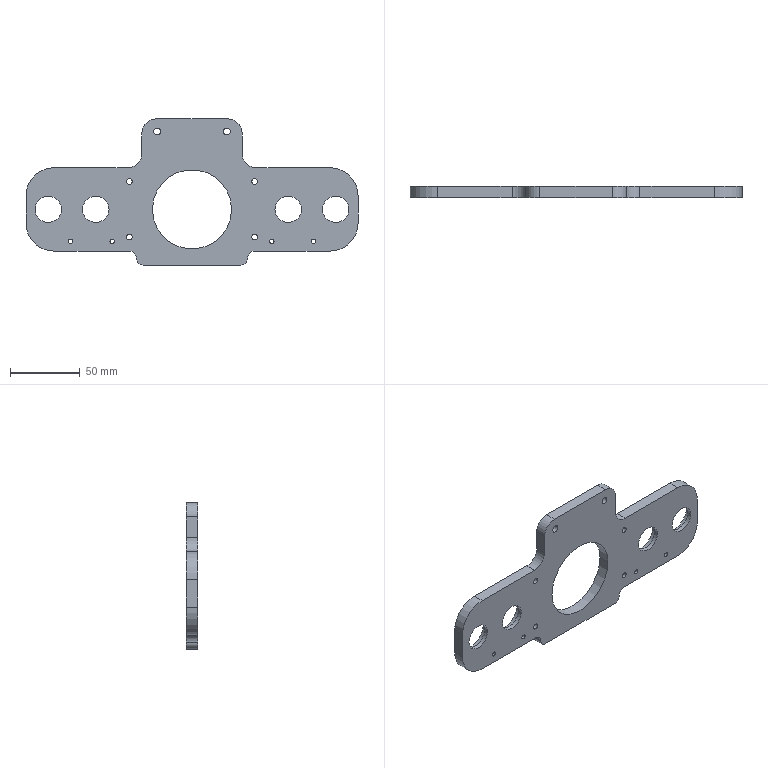Component | SolidWorks | LatestLowerBaseFrame-1 | 1 solid | 84 faces | volume 101960 mm3 | cylinder 62 | plane 22 | commonest cylinder face diameters 4 x8 26 x8 7.5 x8 10 x8 3.2 x8 19 x8 5 x4 20 x4 | material 6061 Alloy